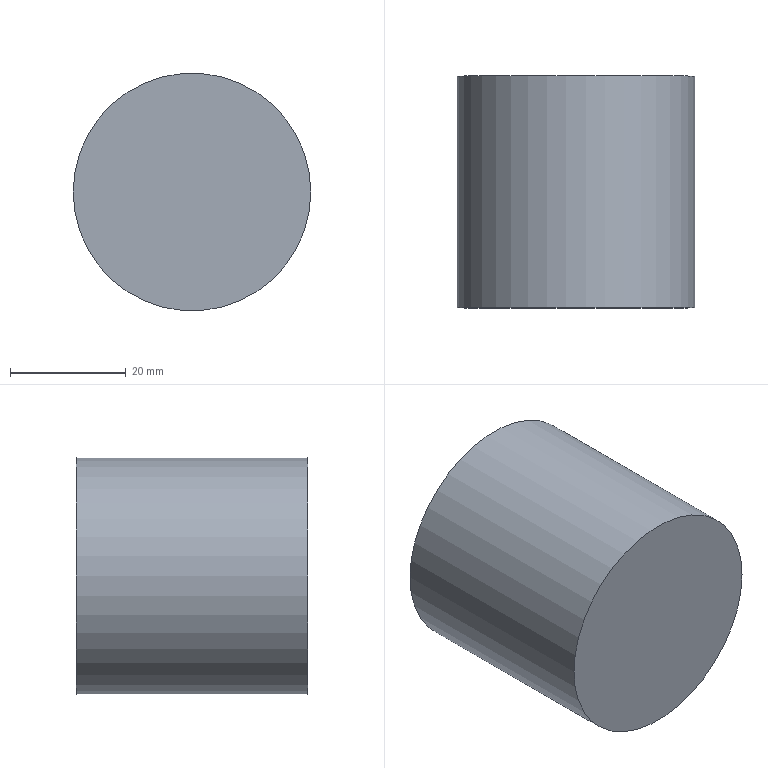Component | NX | MODEL4 | 1 solid | 3 faces | box 41 x 40 x 41 mm | volume 52810 mm3 | plane 2 | cylinder 1 | commonest cylinder face diameters 41 x1
STEP:
#1=CARTESIAN_POINT('',(0.,0.,0.));
#2=DIRECTION('',(0.,0.,1.));
#3=DIRECTION('',(1.,0.,0.));
#4=AXIS2_PLACEMENT_3D('',#1,#2,#3);
#5=CARTESIAN_POINT('',(955.706,15.431,-192.391));
#6=VERTEX_POINT('',#5);
#7=CARTESIAN_POINT('',(935.206,15.431,-192.391));
#8=DIRECTION('',(0.,1.,0.));
#9=DIRECTION('',(1.,0.,0.));
#10=AXIS2_PLACEMENT_3D('',#7,#8,#9);
#11=CIRCLE('',#10,20.5);
#12=CARTESIAN_POINT('',(935.206,15.431,-192.391));
#13=DIRECTION('',(0.,-1.,0.));
#14=DIRECTION('',(-1.,0.,0.));
#15=AXIS2_PLACEMENT_3D('',#12,#13,#14);
#16=CYLINDRICAL_SURFACE('',#15,20.5);
#17=CARTESIAN_POINT('',(9.425,0.));
#18=DIRECTION('',(-1.,0.));
#19=VECTOR('',#18,1.);
#20=LINE('',#17,#19);
#21=(GEOMETRIC_REPRESENTATION_CONTEXT(2)PARAMETRIC_REPRESENTATION_CONTEXT()REPRESENTATION_CONTEXT('',''));
#22=DEFINITIONAL_REPRESENTATION('',(#20),#21);
#23=PCURVE('',#16,#22);
#24=CARTESIAN_POINT('',(935.206,15.431,-192.391));
#25=DIRECTION('',(0.,1.,0.));
#26=DIRECTION('',(1.,0.,0.));
#27=AXIS2_PLACEMENT_3D('',#24,#25,#26);
#28=PLANE('',#27);
#29=CARTESIAN_POINT('',(0.,0.));
#30=DIRECTION('',(1.,0.));
#31=AXIS2_PLACEMENT_2D('',#29,#30);
#32=CIRCLE('',#31,20.5);
#33=(GEOMETRIC_REPRESENTATION_CONTEXT(2)PARAMETRIC_REPRESENTATION_CONTEXT()REPRESENTATION_CONTEXT('',''));
#34=DEFINITIONAL_REPRESENTATION('',(#32),#33);
#35=PCURVE('',#28,#34);
#36=SURFACE_CURVE('',#11,(#23,#35),.PCURVE_S1.);
#37=EDGE_CURVE('',#6,#6,#36,.T.);
#38=ORIENTED_EDGE('',*,*,#37,.F.);
#39=CARTESIAN_POINT('',(955.706,-24.569,-192.391));
#40=VERTEX_POINT('',#39);
#41=CARTESIAN_POINT('',(955.706,15.431,-192.391));
#42=CARTESIAN_POINT('',(955.706,-24.569,-192.391));
#43=B_SPLINE_CURVE_WITH_KNOTS('',1,(#41,#42),.UNSPECIFIED.,.F.,.F.,(2,2),(0.,40.),.PIECEWISE_BEZIER_KNOTS.);
#44=CARTESIAN_POINT('',(9.425,0.));
#45=DIRECTION('',(0.,1.));
#46=VECTOR('',#45,1.);
#47=LINE('',#44,#46);
#48=(GEOMETRIC_REPRESENTATION_CONTEXT(2)PARAMETRIC_REPRESENTATION_CONTEXT()REPRESENTATION_CONTEXT('',''));
#49=DEFINITIONAL_REPRESENTATION('',(#47),#48);
#50=PCURVE('',#16,#49);
#51=CARTESIAN_POINT('',(3.142,0.));
#52=DIRECTION('',(0.,1.));
#53=VECTOR('',#52,1.);
#54=LINE('',#51,#53);
#55=(GEOMETRIC_REPRESENTATION_CONTEXT(2)PARAMETRIC_REPRESENTATION_CONTEXT()REPRESENTATION_CONTEXT('',''));
#56=DEFINITIONAL_REPRESENTATION('',(#54),#55);
#57=PCURVE('',#16,#56);
#58=SEAM_CURVE('',#43,(#50,#57),.PCURVE_S1.);
#59=EDGE_CURVE('',#6,#40,#58,.T.);
#60=ORIENTED_EDGE('',*,*,#59,.T.);
#61=CARTESIAN_POINT('',(935.206,-24.569,-192.391));
#62=DIRECTION('',(0.,1.,0.));
#63=DIRECTION('',(1.,0.,0.));
#64=AXIS2_PLACEMENT_3D('',#61,#62,#63);
#65=CIRCLE('',#64,20.5);
#66=CARTESIAN_POINT('',(9.425,40.));
#67=DIRECTION('',(-1.,0.));
#68=VECTOR('',#67,1.);
#69=LINE('',#66,#68);
#70=(GEOMETRIC_REPRESENTATION_CONTEXT(2)PARAMETRIC_REPRESENTATION_CONTEXT()REPRESENTATION_CONTEXT('',''));
#71=DEFINITIONAL_REPRESENTATION('',(#69),#70);
#72=PCURVE('',#16,#71);
#73=CARTESIAN_POINT('',(935.206,-24.569,-192.391));
#74=DIRECTION('',(0.,1.,0.));
#75=DIRECTION('',(1.,0.,0.));
#76=AXIS2_PLACEMENT_3D('',#73,#74,#75);
#77=PLANE('',#76);
#78=CARTESIAN_POINT('',(0.,0.));
#79=DIRECTION('',(1.,0.));
#80=AXIS2_PLACEMENT_2D('',#78,#79);
#81=CIRCLE('',#80,20.5);
#82=(GEOMETRIC_REPRESENTATION_CONTEXT(2)PARAMETRIC_REPRESENTATION_CONTEXT()REPRESENTATION_CONTEXT('',''));
#83=DEFINITIONAL_REPRESENTATION('',(#81),#82);
#84=PCURVE('',#77,#83);
#85=SURFACE_CURVE('',#65,(#72,#84),.PCURVE_S1.);
#86=EDGE_CURVE('',#40,#40,#85,.T.);
#87=ORIENTED_EDGE('',*,*,#86,.T.);
#88=ORIENTED_EDGE('',*,*,#59,.F.);
#89=EDGE_LOOP('',(#38,#60,#87,#88));
#90=FACE_BOUND('',#89,.T.);
#91=ADVANCED_FACE('',(#90),#16,.T.);
#92=ORIENTED_EDGE('',*,*,#37,.T.);
#93=EDGE_LOOP('',(#92));
#94=FACE_BOUND('',#93,.T.);
#95=ADVANCED_FACE('',(#94),#28,.T.);
#96=ORIENTED_EDGE('',*,*,#86,.F.);
#97=EDGE_LOOP('',(#96));
#98=FACE_BOUND('',#97,.T.);
#99=ADVANCED_FACE('',(#98),#77,.F.);
#100=CLOSED_SHELL('',(#91,#95,#99));
#101=MANIFOLD_SOLID_BREP('',#100);
#102=(LENGTH_UNIT()NAMED_UNIT(*)SI_UNIT(.MILLI.,.METRE.));
#103=UNCERTAINTY_MEASURE_WITH_UNIT(LENGTH_MEASURE(0.00001),#102,'','');
#104=(NAMED_UNIT(*)PLANE_ANGLE_UNIT()SI_UNIT($,.RADIAN.));
#105=(NAMED_UNIT(*)SI_UNIT($,.STERADIAN.)SOLID_ANGLE_UNIT());
#106=(GEOMETRIC_REPRESENTATION_CONTEXT(3)GLOBAL_UNCERTAINTY_ASSIGNED_CONTEXT((#103))GLOBAL_UNIT_ASSIGNED_CONTEXT((#102,#104,#105))REPRESENTATION_CONTEXT('',''));
#107=ADVANCED_BREP_SHAPE_REPRESENTATION('',(#4,#101),#106);